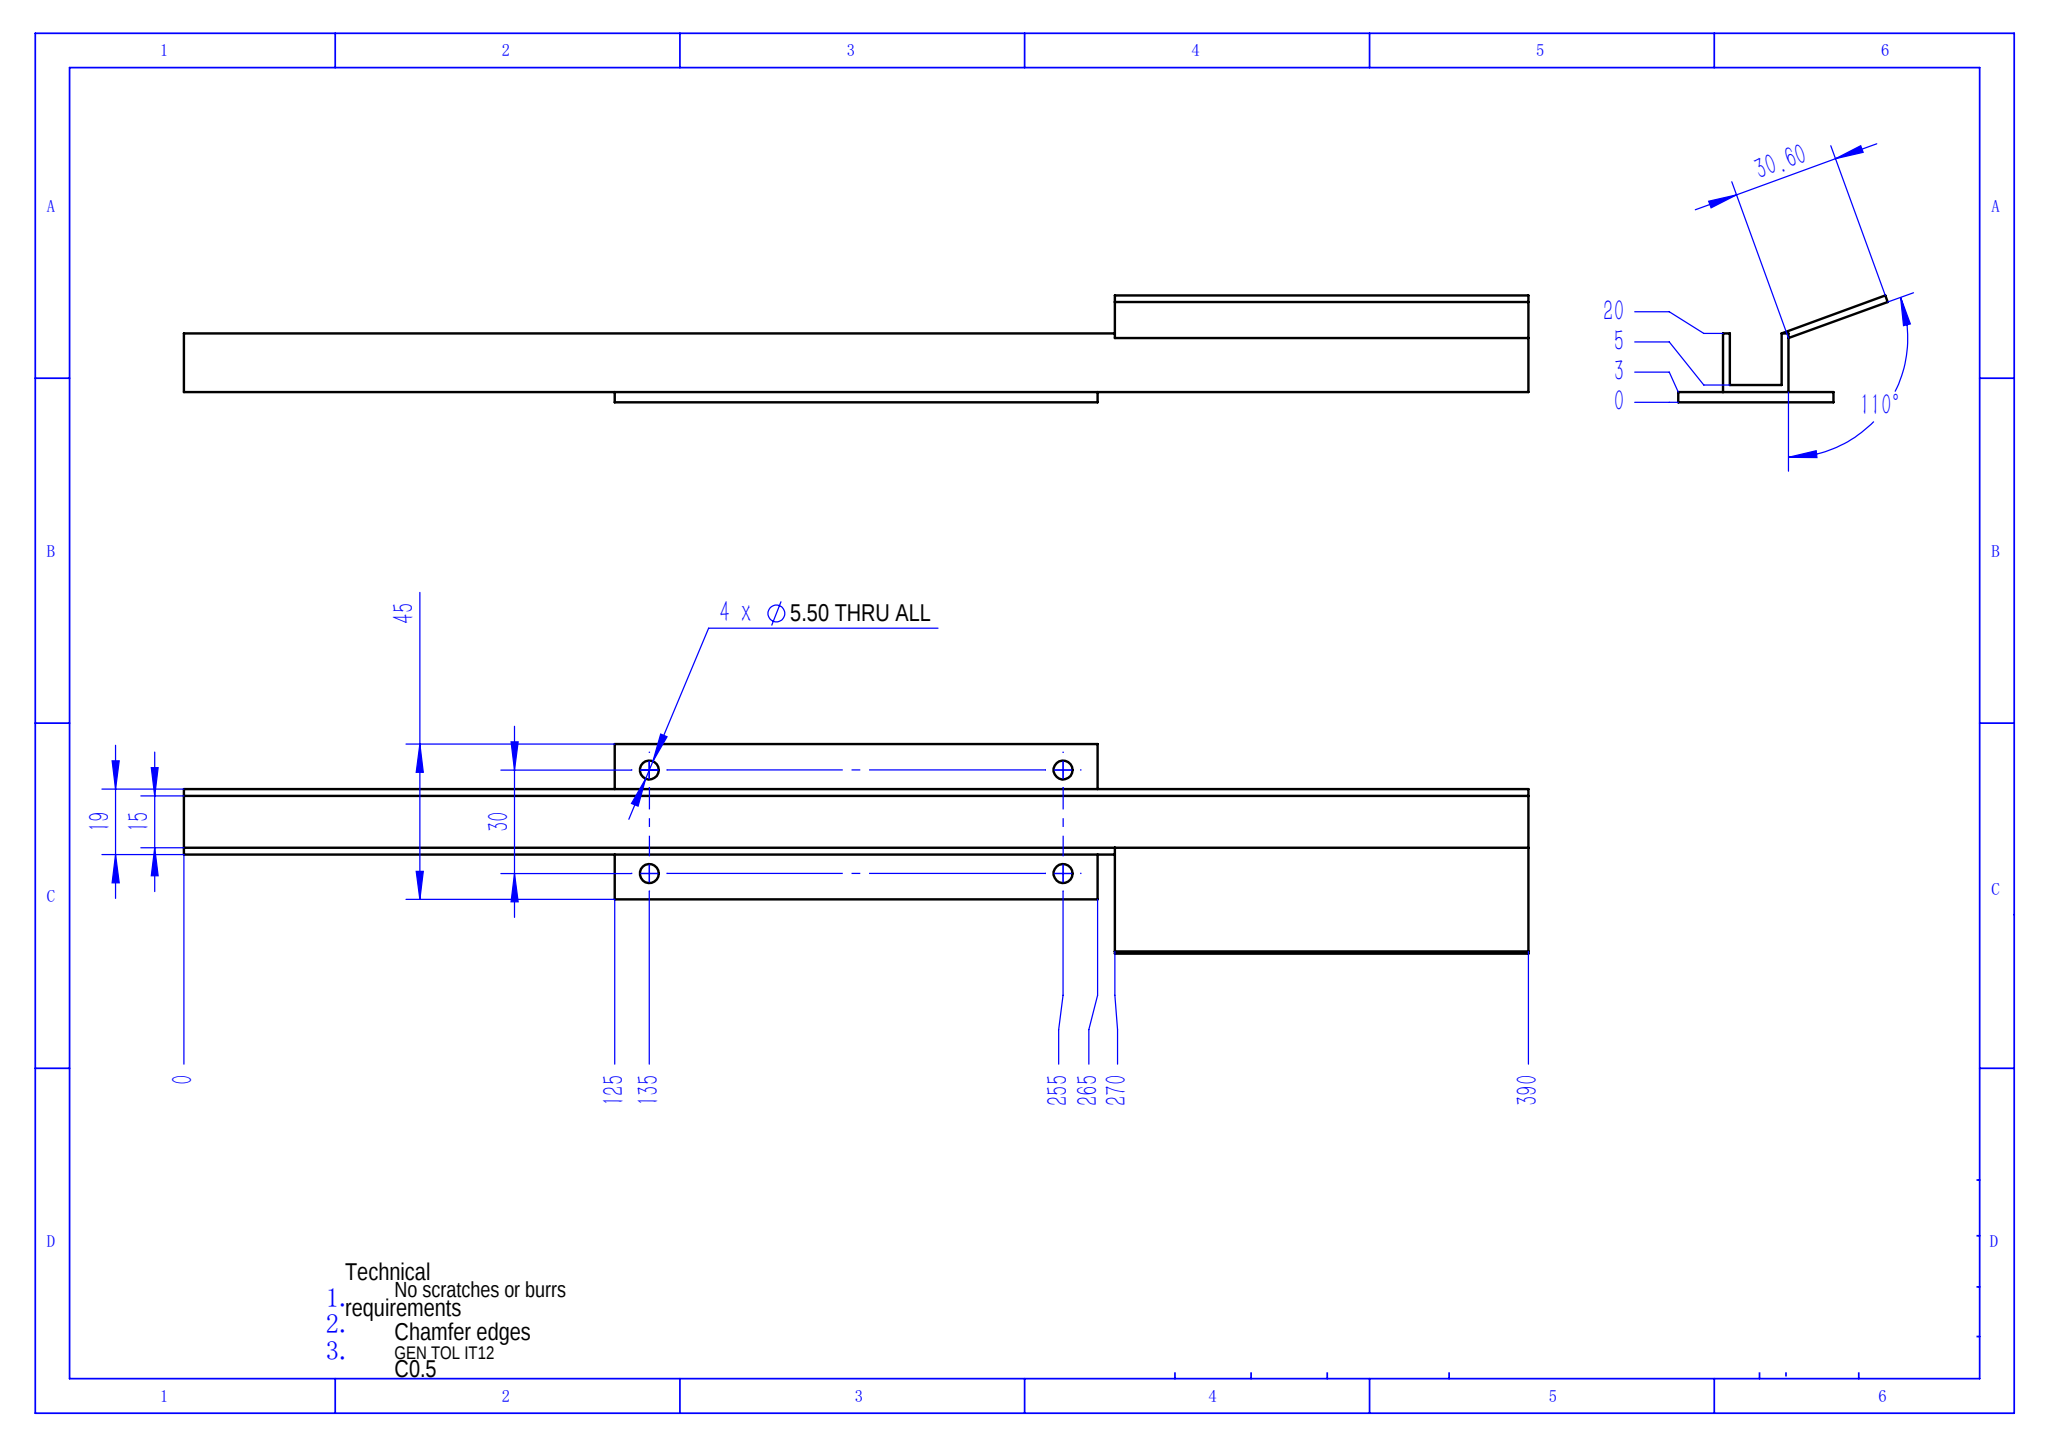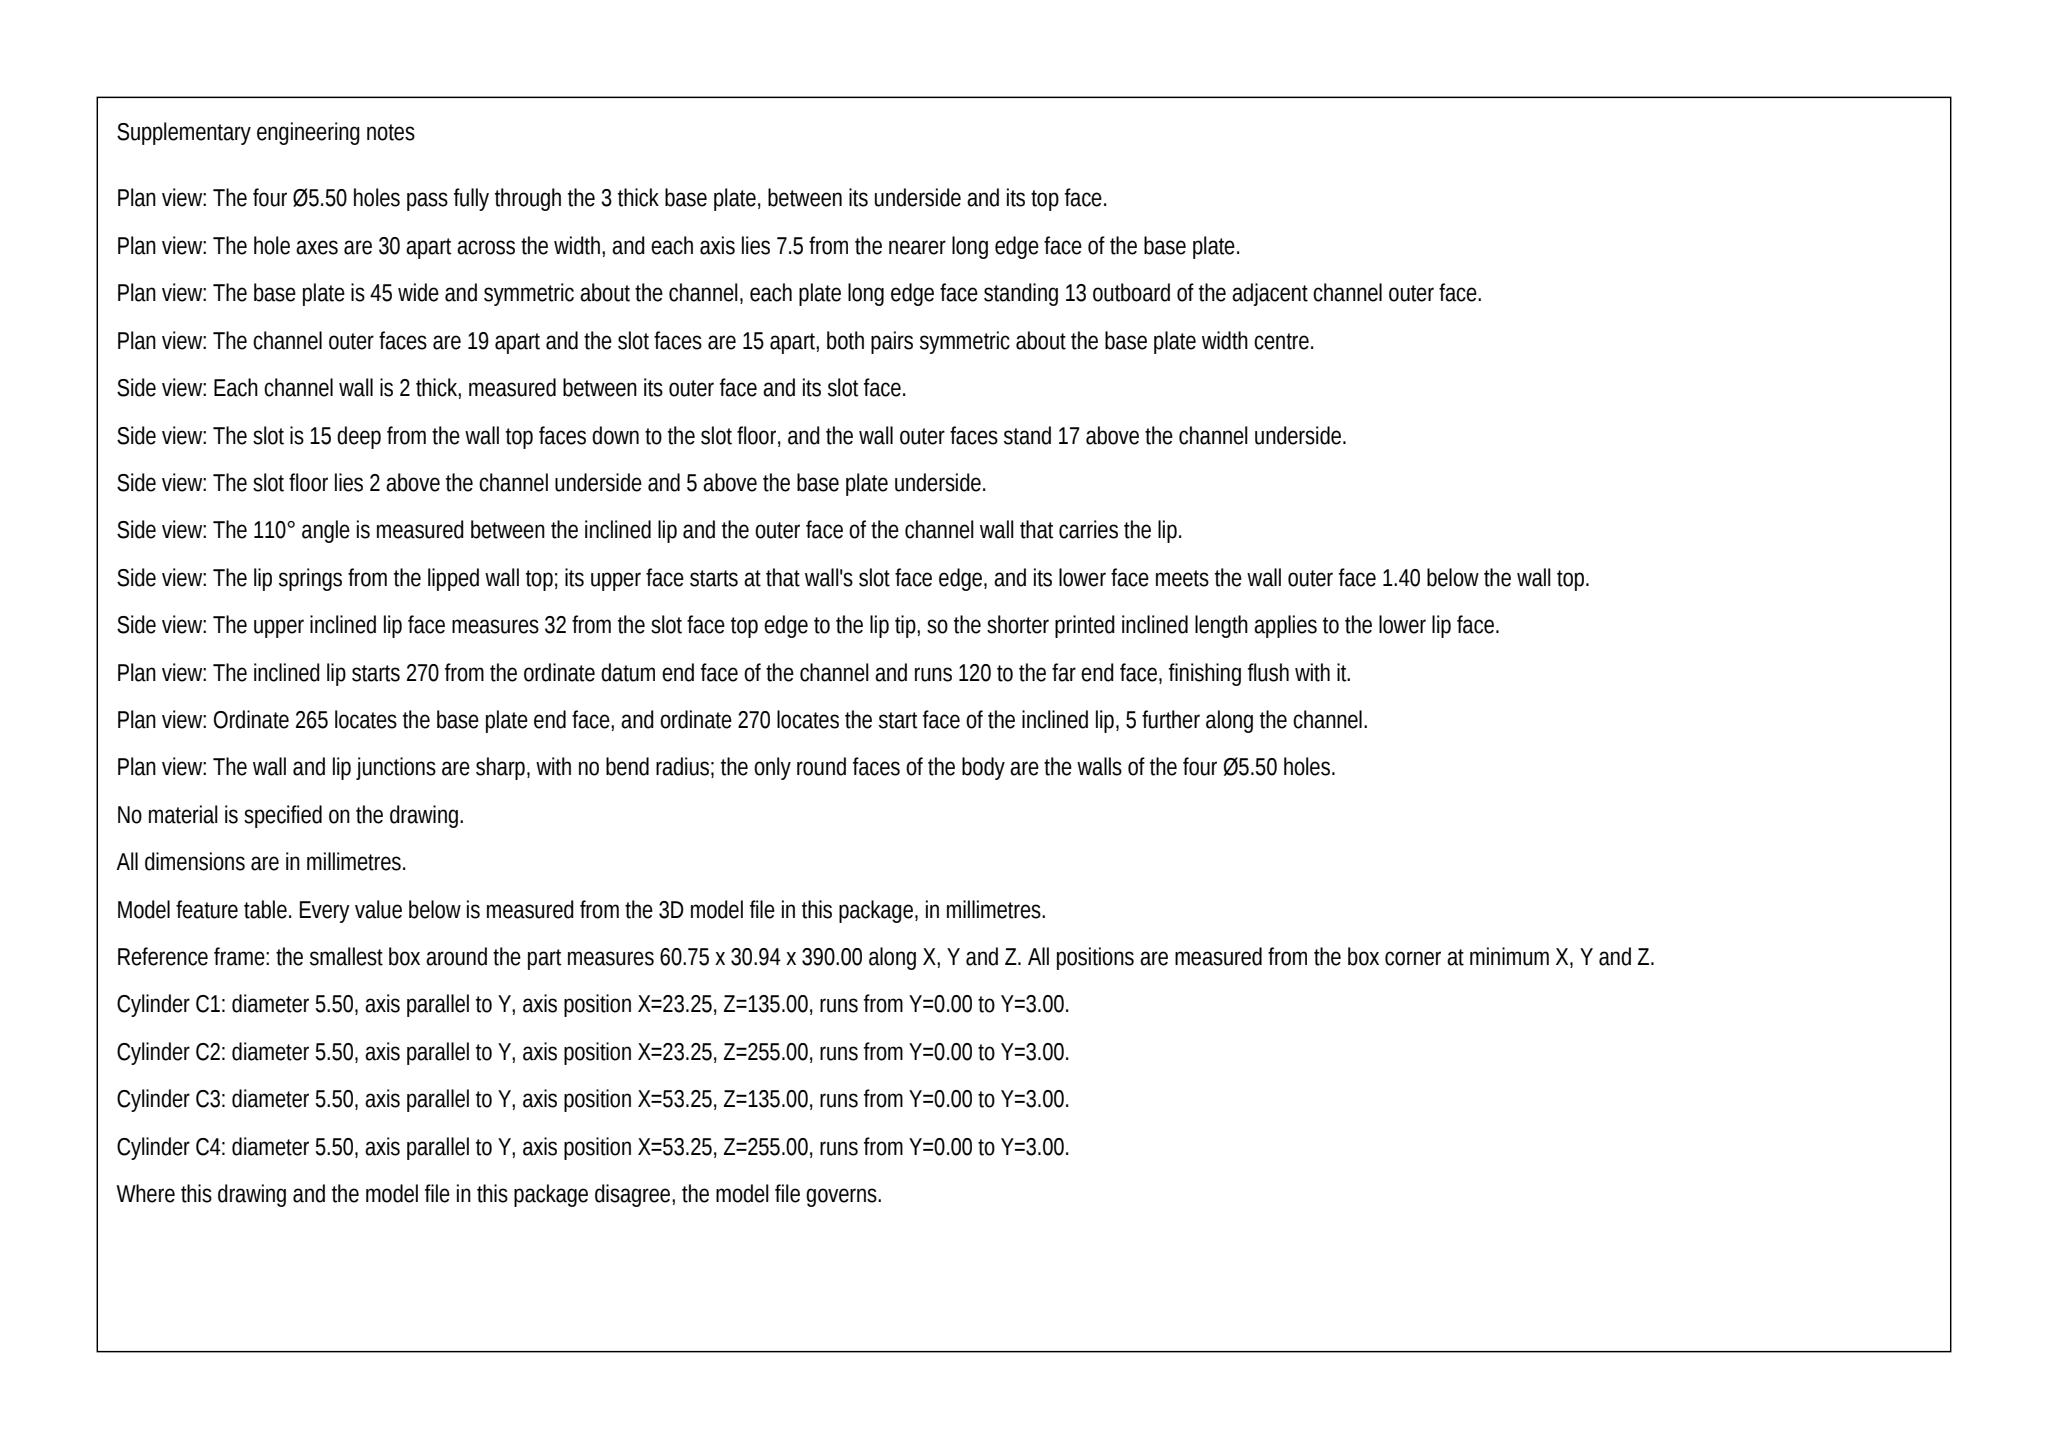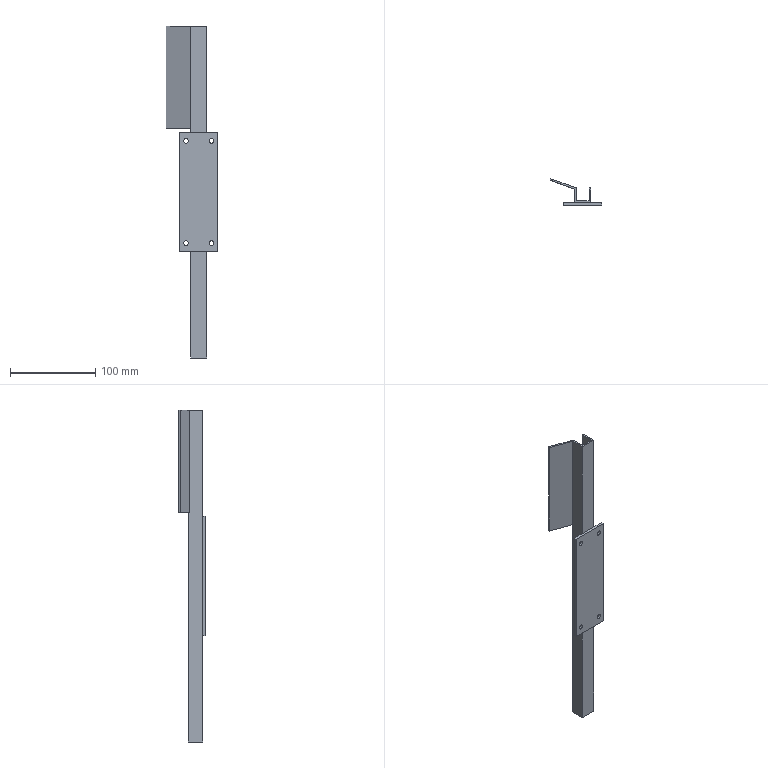Part | SolidWorks | mm | 1 solid | 30 faces | box 60.75 x 30.94 x 390 mm | volume 64179 mm3 | plane 22 | cylinder 8 | commonest cylinder face diameters 5.5 x8
Drawing notes:
110° BENT LIP: 2 THK (30.60 LG FACE) | from the solid: Flange outer face L=28.75/cos20=30.595≈30.60; offset 2 perp gives inner face start at y=20 (wall top plane) and tip at bbox x_min=0, y_max=30.945; matches 2 mm wall thk (x planes 28.75/30.75)
build123d program:
from build123d import *

# Parameters (mm, degrees)
BOSS_EXTRUDE1_DEPTH      = 195
BOSS_EXTRUDE1_DEPTH_BACK = 195
SKETCH2_W                = 45
SKETCH2_H                = 140
BOSS_EXTRUDE2_DEPTH      = 3
M5_CLEARANCE_HOLE1_D     = 5.5
BOSS_EXTRUDE3_DEPTH      = 120


with BuildPart() as part:
    # Sketch1 → Boss-Extrude1 (new, two sides: drawn at the far end of the back side and taken through both)
    with BuildSketch(Plane.XY.offset(-BOSS_EXTRUDE1_DEPTH_BACK)):
        Polygon((7.5, 17), (9.5, 17), (9.5, 0), (-9.5, 0), (-9.5, 17), (-7.5, 17), (-7.5, 2), (7.5, 2), align=None)
    extrude(amount=BOSS_EXTRUDE1_DEPTH + BOSS_EXTRUDE1_DEPTH_BACK)

    # Sketch2 → Boss-Extrude2 (add)
    with BuildSketch(Plane(origin=(0, 0, 0), x_dir=(1, 0, 0), z_dir=(0, 1, 0))):
        Rectangle(SKETCH2_W, SKETCH2_H)
    extrude(amount=-BOSS_EXTRUDE2_DEPTH)

    # M5 Clearance Hole1 (through all)
    with Locations(Plane(origin=(0, 0, 0), x_dir=(1, 0, 0), z_dir=(0, 1, 0))):
        with Locations((-15, 60), (15, -60), (-15, -60), (15, 60)):
            Hole(M5_CLEARANCE_HOLE1_D / 2)

    # Sketch5 → Boss-Extrude3 (add)
    with BuildSketch(Plane.XY.offset(195)):
        Polygon((-7.5, 17), (-8.184, 15.121), (-38.254, 26.065), (-37.57, 27.945), align=None)
    extrude(amount=-BOSS_EXTRUDE3_DEPTH)


solid = part.part